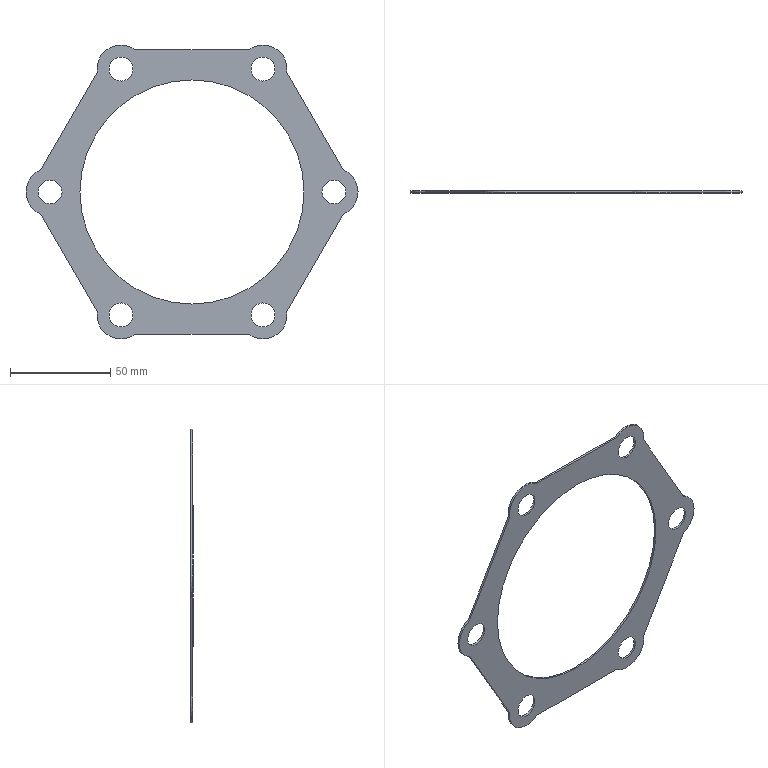Component | NX | T1_SHIM3 | 1 solid | 21 faces | volume 7220 mm3 | cylinder 13 | plane 8 | commonest cylinder face diameters 24 x6 12 x6 112 x1